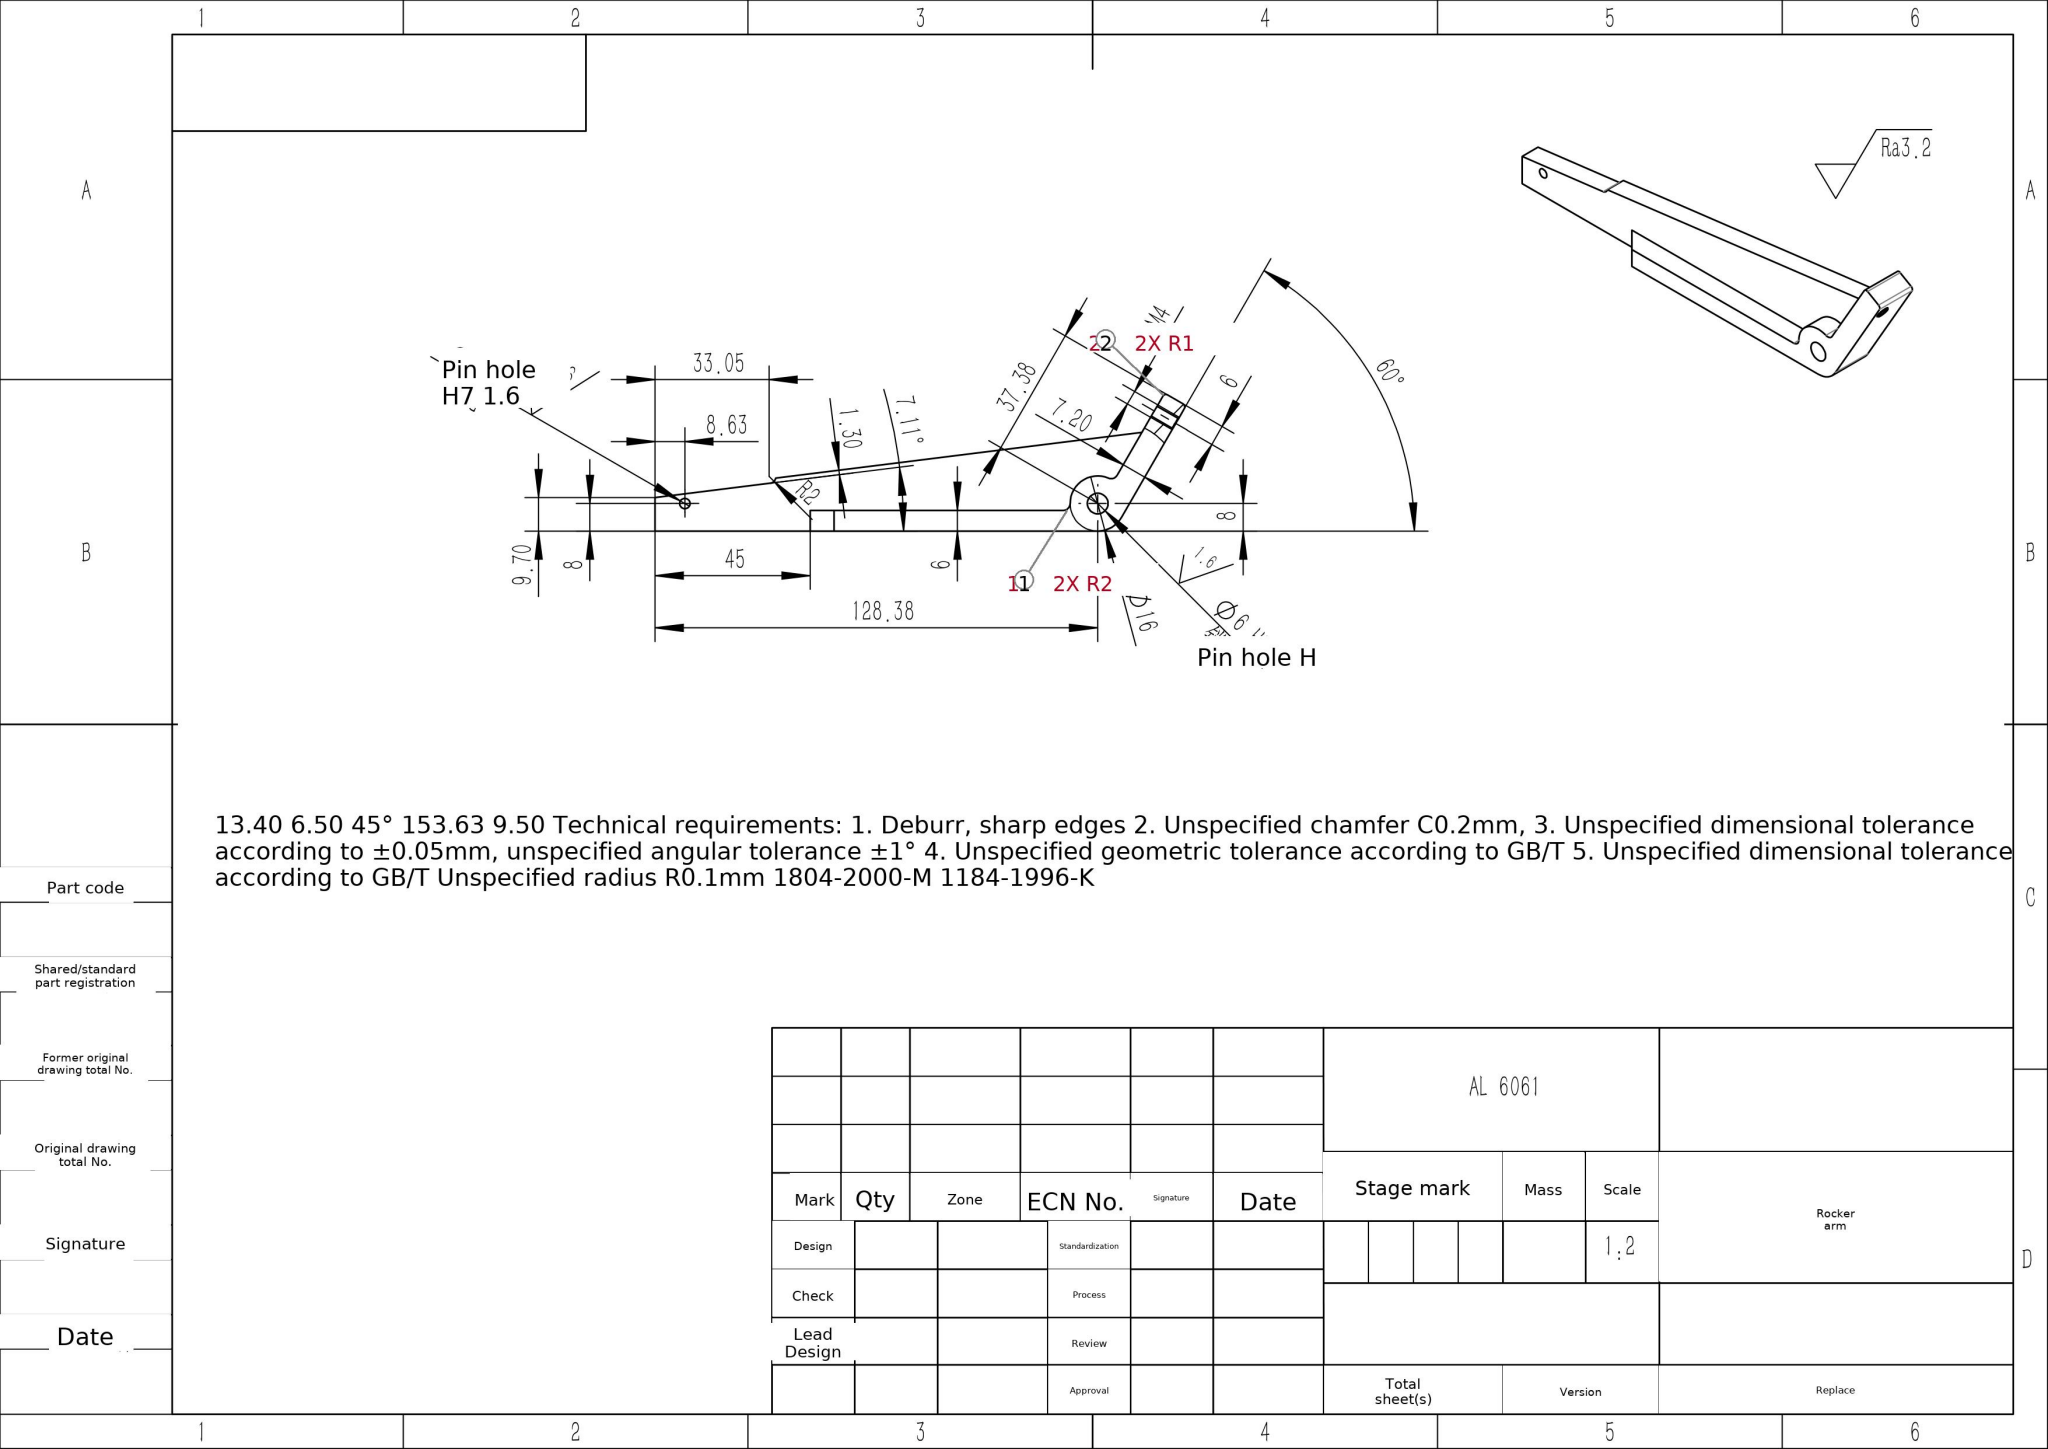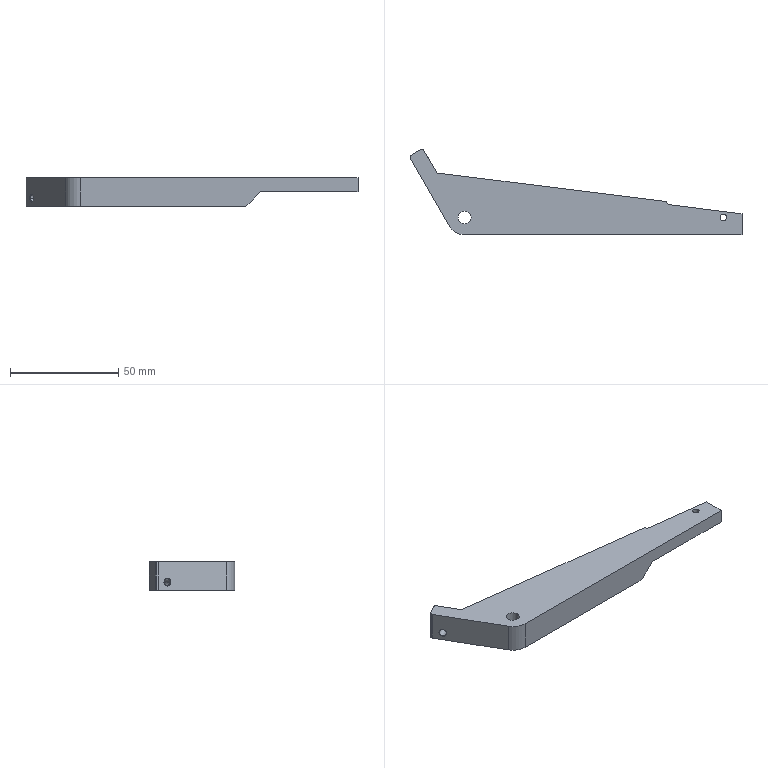Part | SolidWorks | mm | material AL 6061 | 1 solid | 28 faces | box 153.63 x 39.61 x 13.4 mm | volume 23931 mm3 | cylinder 14 | plane 12 | cone 2 | commonest cylinder face diameters 2 x3 4 x3 3.3 x2 6 x2 3 x2 16 x2
STEP:
#1=CARTESIAN_POINT('',(-89.039,32.706,-3.));
#2=VERTEX_POINT('',#1);
#3=CARTESIAN_POINT('',(-87.389,29.848,-3.));
#4=VERTEX_POINT('',#3);
#5=CARTESIAN_POINT('',(-88.214,31.277,-3.));
#6=DIRECTION('',(-0.866,-0.5,0.));
#7=DIRECTION('',(-0.5,0.866,0.));
#8=AXIS2_PLACEMENT_3D('',#5,#6,#7);
#9=CIRCLE('',#8,1.65);
#10=EDGE_CURVE('',#2,#4,#9,.T.);
#11=ORIENTED_EDGE('',*,*,#10,.F.);
#12=CARTESIAN_POINT('',(-89.312,32.779,-3.));
#13=VERTEX_POINT('',#12);
#14=CARTESIAN_POINT('',(-89.039,32.706,-3.));
#15=DIRECTION('',(-0.9659,0.2588,0.));
#16=VECTOR('',#15,1000.);
#17=LINE('',#14,#16);
#18=EDGE_CURVE('',#2,#13,#17,.T.);
#19=ORIENTED_EDGE('',*,*,#18,.T.);
#20=CARTESIAN_POINT('',(-87.462,29.575,-3.));
#21=VERTEX_POINT('',#20);
#22=CARTESIAN_POINT('',(-88.387,31.177,-3.));
#23=DIRECTION('',(0.866,0.5,0.));
#24=DIRECTION('',(-0.5,0.866,0.));
#25=AXIS2_PLACEMENT_3D('',#22,#23,#24);
#26=CIRCLE('',#25,1.85);
#27=EDGE_CURVE('',#21,#13,#26,.T.);
#28=ORIENTED_EDGE('',*,*,#27,.F.);
#29=CARTESIAN_POINT('',(-87.389,29.848,-3.));
#30=DIRECTION('',(-0.2588,-0.9659,0.));
#31=VECTOR('',#30,1000.);
#32=LINE('',#29,#31);
#33=EDGE_CURVE('',#4,#21,#32,.T.);
#34=ORIENTED_EDGE('',*,*,#33,.F.);
#35=EDGE_LOOP('',(#11,#19,#28,#34));
#36=FACE_OUTER_BOUND('',#35,.T.);
#37=CARTESIAN_POINT('',(-88.214,31.277,-3.));
#38=DIRECTION('',(-0.866,-0.5,0.));
#39=DIRECTION('',(0.5,-0.866,0.));
#40=AXIS2_PLACEMENT_3D('',#37,#38,#39);
#41=CONICAL_SURFACE('',#40,1.65,0.7854);
#42=ADVANCED_FACE('',(#36),#41,.F.);
#43=CARTESIAN_POINT('',(-82.976,36.206,-3.));
#44=VERTEX_POINT('',#43);
#45=CARTESIAN_POINT('',(-81.326,33.348,-3.));
#46=VERTEX_POINT('',#45);
#47=CARTESIAN_POINT('',(-82.151,34.777,-3.));
#48=DIRECTION('',(-0.866,-0.5,0.));
#49=DIRECTION('',(0.5,-0.866,0.));
#50=AXIS2_PLACEMENT_3D('',#47,#48,#49);
#51=CIRCLE('',#50,1.65);
#52=EDGE_CURVE('',#44,#46,#51,.T.);
#53=ORIENTED_EDGE('',*,*,#52,.F.);
#54=CARTESIAN_POINT('',(27.688,100.098,-3.));
#55=DIRECTION('',(-0.866,-0.5,0.));
#56=VECTOR('',#55,1000.);
#57=LINE('',#54,#56);
#58=EDGE_CURVE('',#44,#2,#57,.T.);
#59=ORIENTED_EDGE('',*,*,#58,.T.);
#60=ORIENTED_EDGE('',*,*,#10,.T.);
#61=CARTESIAN_POINT('',(29.338,97.24,-3.));
#62=DIRECTION('',(-0.866,-0.5,0.));
#63=VECTOR('',#62,1000.);
#64=LINE('',#61,#63);
#65=EDGE_CURVE('',#46,#4,#64,.T.);
#66=ORIENTED_EDGE('',*,*,#65,.F.);
#67=EDGE_LOOP('',(#53,#59,#60,#66));
#68=FACE_OUTER_BOUND('',#67,.T.);
#69=CARTESIAN_POINT('',(28.513,98.669,-3.));
#70=DIRECTION('',(-0.866,-0.5,0.));
#71=DIRECTION('',(0.5,-0.866,0.));
#72=AXIS2_PLACEMENT_3D('',#69,#70,#71);
#73=CYLINDRICAL_SURFACE('',#72,1.65);
#74=ADVANCED_FACE('',(#68),#73,.F.);
#75=CARTESIAN_POINT('',(-62.768,8.,-6.9));
#76=VERTEX_POINT('',#75);
#77=CARTESIAN_POINT('',(-68.768,8.,-6.9));
#78=VERTEX_POINT('',#77);
#79=CARTESIAN_POINT('',(-65.768,8.,-6.9));
#80=DIRECTION('',(0.,0.,-1.));
#81=DIRECTION('',(1.,0.,0.));
#82=AXIS2_PLACEMENT_3D('',#79,#80,#81);
#83=CIRCLE('',#82,3.);
#84=EDGE_CURVE('',#76,#78,#83,.T.);
#85=ORIENTED_EDGE('',*,*,#84,.T.);
#86=CARTESIAN_POINT('',(-68.768,8.,6.5));
#87=VERTEX_POINT('',#86);
#88=CARTESIAN_POINT('',(-68.768,8.,-15.485));
#89=DIRECTION('',(0.,0.,1.));
#90=VECTOR('',#89,1000.);
#91=LINE('',#88,#90);
#92=EDGE_CURVE('',#78,#87,#91,.T.);
#93=ORIENTED_EDGE('',*,*,#92,.T.);
#94=CARTESIAN_POINT('',(-62.768,8.,6.5));
#95=VERTEX_POINT('',#94);
#96=CARTESIAN_POINT('',(-65.768,8.,6.5));
#97=DIRECTION('',(0.,0.,1.));
#98=DIRECTION('',(1.,0.,0.));
#99=AXIS2_PLACEMENT_3D('',#96,#97,#98);
#100=CIRCLE('',#99,3.);
#101=EDGE_CURVE('',#87,#95,#100,.T.);
#102=ORIENTED_EDGE('',*,*,#101,.T.);
#103=CARTESIAN_POINT('',(-62.768,8.,-15.485));
#104=DIRECTION('',(0.,0.,1.));
#105=VECTOR('',#104,1000.);
#106=LINE('',#103,#105);
#107=EDGE_CURVE('',#76,#95,#106,.T.);
#108=ORIENTED_EDGE('',*,*,#107,.F.);
#109=EDGE_LOOP('',(#85,#93,#102,#108));
#110=FACE_OUTER_BOUND('',#109,.T.);
#111=CARTESIAN_POINT('',(-65.768,8.,-15.485));
#112=DIRECTION('',(0.,0.,1.));
#113=DIRECTION('',(1.,0.,0.));
#114=AXIS2_PLACEMENT_3D('',#111,#112,#113);
#115=CYLINDRICAL_SURFACE('',#114,3.);
#116=ADVANCED_FACE('',(#110),#115,.F.);
#117=CARTESIAN_POINT('',(-91.021,36.007,6.5));
#118=VERTEX_POINT('',#117);
#119=CARTESIAN_POINT('',(-90.887,35.507,6.5));
#120=VERTEX_POINT('',#119);
#121=CARTESIAN_POINT('',(-90.021,36.007,6.5));
#122=DIRECTION('',(0.,0.,1.));
#123=DIRECTION('',(1.,0.,0.));
#124=AXIS2_PLACEMENT_3D('',#121,#122,#123);
#125=CIRCLE('',#124,1.);
#126=EDGE_CURVE('',#118,#120,#125,.T.);
#127=ORIENTED_EDGE('',*,*,#126,.F.);
#128=CARTESIAN_POINT('',(-91.021,36.007,-6.9));
#129=VERTEX_POINT('',#128);
#130=CARTESIAN_POINT('',(-91.021,36.007,6.5));
#131=DIRECTION('',(0.,0.,-1.));
#132=VECTOR('',#131,1000.);
#133=LINE('',#130,#132);
#134=EDGE_CURVE('',#118,#129,#133,.T.);
#135=ORIENTED_EDGE('',*,*,#134,.T.);
#136=CARTESIAN_POINT('',(-90.887,35.507,-6.9));
#137=VERTEX_POINT('',#136);
#138=CARTESIAN_POINT('',(-90.021,36.007,-6.9));
#139=DIRECTION('',(0.,0.,1.));
#140=DIRECTION('',(1.,0.,0.));
#141=AXIS2_PLACEMENT_3D('',#138,#139,#140);
#142=CIRCLE('',#141,1.);
#143=EDGE_CURVE('',#129,#137,#142,.T.);
#144=ORIENTED_EDGE('',*,*,#143,.T.);
#145=CARTESIAN_POINT('',(-90.887,35.507,6.5));
#146=DIRECTION('',(0.,0.,-1.));
#147=VECTOR('',#146,1000.);
#148=LINE('',#145,#147);
#149=EDGE_CURVE('',#120,#137,#148,.T.);
#150=ORIENTED_EDGE('',*,*,#149,.F.);
#151=EDGE_LOOP('',(#127,#135,#144,#150));
#152=FACE_OUTER_BOUND('',#151,.T.);
#153=CARTESIAN_POINT('',(-90.021,36.007,6.5));
#154=DIRECTION('',(0.,0.,-1.));
#155=DIRECTION('',(-1.,0.,0.));
#156=AXIS2_PLACEMENT_3D('',#153,#154,#155);
#157=CYLINDRICAL_SURFACE('',#156,1.);
#158=ADVANCED_FACE('',(#152),#157,.T.);
#159=CARTESIAN_POINT('',(52.482,8.,0.));
#160=VERTEX_POINT('',#159);
#161=CARTESIAN_POINT('',(55.482,8.,0.));
#162=VERTEX_POINT('',#161);
#163=CARTESIAN_POINT('',(53.982,8.,0.));
#164=DIRECTION('',(0.,0.,1.));
#165=DIRECTION('',(1.,0.,0.));
#166=AXIS2_PLACEMENT_3D('',#163,#164,#165);
#167=CIRCLE('',#166,1.5);
#168=EDGE_CURVE('',#160,#162,#167,.T.);
#169=ORIENTED_EDGE('',*,*,#168,.F.);
#170=CARTESIAN_POINT('',(52.482,8.,6.5));
#171=VERTEX_POINT('',#170);
#172=CARTESIAN_POINT('',(52.482,8.,-0.5));
#173=DIRECTION('',(0.,0.,1.));
#174=VECTOR('',#173,1000.);
#175=LINE('',#172,#174);
#176=EDGE_CURVE('',#160,#171,#175,.T.);
#177=ORIENTED_EDGE('',*,*,#176,.T.);
#178=CARTESIAN_POINT('',(55.482,8.,6.5));
#179=VERTEX_POINT('',#178);
#180=CARTESIAN_POINT('',(53.982,8.,6.5));
#181=DIRECTION('',(0.,0.,1.));
#182=DIRECTION('',(1.,0.,0.));
#183=AXIS2_PLACEMENT_3D('',#180,#181,#182);
#184=CIRCLE('',#183,1.5);
#185=EDGE_CURVE('',#171,#179,#184,.T.);
#186=ORIENTED_EDGE('',*,*,#185,.T.);
#187=CARTESIAN_POINT('',(55.482,8.,-0.5));
#188=DIRECTION('',(0.,0.,1.));
#189=VECTOR('',#188,1000.);
#190=LINE('',#187,#189);
#191=EDGE_CURVE('',#162,#179,#190,.T.);
#192=ORIENTED_EDGE('',*,*,#191,.F.);
#193=EDGE_LOOP('',(#169,#177,#186,#192));
#194=FACE_OUTER_BOUND('',#193,.T.);
#195=CARTESIAN_POINT('',(53.982,8.,-0.5));
#196=DIRECTION('',(0.,0.,1.));
#197=DIRECTION('',(1.,0.,0.));
#198=AXIS2_PLACEMENT_3D('',#195,#196,#197);
#199=CYLINDRICAL_SURFACE('',#198,1.5);
#200=ADVANCED_FACE('',(#194),#199,.F.);
#201=CARTESIAN_POINT('',(-82.151,34.777,-3.));
#202=DIRECTION('',(-0.866,-0.5,0.));
#203=DIRECTION('',(0.5,-0.866,0.));
#204=AXIS2_PLACEMENT_3D('',#201,#202,#203);
#205=CIRCLE('',#204,1.65);
#206=EDGE_CURVE('',#46,#44,#205,.T.);
#207=ORIENTED_EDGE('',*,*,#206,.T.);
#208=ORIENTED_EDGE('',*,*,#52,.T.);
#209=EDGE_LOOP('',(#207,#208));
#210=FACE_BOUND('',#209,.T.);
#211=CARTESIAN_POINT('',(-71.425,16.198,0.));
#212=VERTEX_POINT('',#211);
#213=CARTESIAN_POINT('',(-71.425,16.198,-6.9));
#214=VERTEX_POINT('',#213);
#215=CARTESIAN_POINT('',(-71.425,16.198,-7.));
#216=DIRECTION('',(0.,0.,-1.));
#217=VECTOR('',#216,1000.);
#218=LINE('',#215,#217);
#219=EDGE_CURVE('',#212,#214,#218,.T.);
#220=ORIENTED_EDGE('',*,*,#219,.T.);
#221=CARTESIAN_POINT('',(-84.651,39.107,-6.9));
#222=VERTEX_POINT('',#221);
#223=CARTESIAN_POINT('',(-85.151,39.973,-6.9));
#224=DIRECTION('',(-0.5,0.866,0.));
#225=VECTOR('',#224,1000.);
#226=LINE('',#223,#225);
#227=EDGE_CURVE('',#214,#222,#226,.T.);
#228=ORIENTED_EDGE('',*,*,#227,.T.);
#229=CARTESIAN_POINT('',(-84.651,39.107,6.5));
#230=VERTEX_POINT('',#229);
#231=CARTESIAN_POINT('',(-84.651,39.107,6.5));
#232=DIRECTION('',(0.,0.,1.));
#233=VECTOR('',#232,1000.);
#234=LINE('',#231,#233);
#235=EDGE_CURVE('',#222,#230,#234,.T.);
#236=ORIENTED_EDGE('',*,*,#235,.T.);
#237=CARTESIAN_POINT('',(-78.598,28.621,6.5));
#238=VERTEX_POINT('',#237);
#239=CARTESIAN_POINT('',(-85.151,39.973,6.5));
#240=DIRECTION('',(-0.5,0.866,0.));
#241=VECTOR('',#240,1000.);
#242=LINE('',#239,#241);
#243=EDGE_CURVE('',#238,#230,#242,.T.);
#244=ORIENTED_EDGE('',*,*,#243,.F.);
#245=CARTESIAN_POINT('',(-78.598,28.621,0.));
#246=VERTEX_POINT('',#245);
#247=CARTESIAN_POINT('',(-78.598,28.621,6.5));
#248=DIRECTION('',(-0.,-0.,-1.));
#249=VECTOR('',#248,1000.);
#250=LINE('',#247,#249);
#251=EDGE_CURVE('',#238,#246,#250,.T.);
#252=ORIENTED_EDGE('',*,*,#251,.T.);
#253=CARTESIAN_POINT('',(-46.555,-26.878,0.));
#254=DIRECTION('',(0.5,-0.866,0.));
#255=VECTOR('',#254,1000.);
#256=LINE('',#253,#255);
#257=EDGE_CURVE('',#246,#212,#256,.T.);
#258=ORIENTED_EDGE('',*,*,#257,.T.);
#259=EDGE_LOOP('',(#220,#228,#236,#244,#252,#258));
#260=FACE_OUTER_BOUND('',#259,.T.);
#261=CARTESIAN_POINT('',(-85.151,39.973,6.5));
#262=DIRECTION('',(-0.866,-0.5,0.));
#263=DIRECTION('',(0.5,-0.866,0.));
#264=AXIS2_PLACEMENT_3D('',#261,#262,#263);
#265=PLANE('',#264);
#266=ADVANCED_FACE('',(#210,#260),#265,.F.);
#267=CARTESIAN_POINT('',(-55.768,6.,-6.9));
#268=VERTEX_POINT('',#267);
#269=CARTESIAN_POINT('',(-55.768,6.,0.));
#270=VERTEX_POINT('',#269);
#271=CARTESIAN_POINT('',(-55.768,6.,0.));
#272=DIRECTION('',(0.,0.,1.));
#273=VECTOR('',#272,1000.);
#274=LINE('',#271,#273);
#275=EDGE_CURVE('',#268,#270,#274,.T.);
#276=ORIENTED_EDGE('',*,*,#275,.T.);
#277=CARTESIAN_POINT('',(17.613,6.,0.));
#278=VERTEX_POINT('',#277);
#279=CARTESIAN_POINT('',(-0.,6.,0.));
#280=DIRECTION('',(1.,0.,0.));
#281=VECTOR('',#280,1000.);
#282=LINE('',#279,#281);
#283=EDGE_CURVE('',#270,#278,#282,.T.);
#284=ORIENTED_EDGE('',*,*,#283,.T.);
#285=CARTESIAN_POINT('',(10.713,6.,-6.9));
#286=VERTEX_POINT('',#285);
#287=CARTESIAN_POINT('',(10.613,6.,-7.));
#288=DIRECTION('',(-0.7071,-0.,-0.7071));
#289=VECTOR('',#288,1000.);
#290=LINE('',#287,#289);
#291=EDGE_CURVE('',#278,#286,#290,.T.);
#292=ORIENTED_EDGE('',*,*,#291,.T.);
#293=CARTESIAN_POINT('',(-0.,6.,-6.9));
#294=DIRECTION('',(1.,0.,0.));
#295=VECTOR('',#294,1000.);
#296=LINE('',#293,#295);
#297=EDGE_CURVE('',#268,#286,#296,.T.);
#298=ORIENTED_EDGE('',*,*,#297,.F.);
#299=EDGE_LOOP('',(#276,#284,#292,#298));
#300=FACE_OUTER_BOUND('',#299,.T.);
#301=CARTESIAN_POINT('',(17.613,6.,-7.));
#302=DIRECTION('',(0.,-1.,0.));
#303=DIRECTION('',(1.,0.,0.));
#304=AXIS2_PLACEMENT_3D('',#301,#302,#303);
#305=PLANE('',#304);
#306=ADVANCED_FACE('',(#300),#305,.F.);
#307=CARTESIAN_POINT('',(53.982,8.,0.));
#308=DIRECTION('',(0.,0.,1.));
#309=DIRECTION('',(1.,0.,0.));
#310=AXIS2_PLACEMENT_3D('',#307,#308,#309);
#311=CIRCLE('',#310,1.5);
#312=EDGE_CURVE('',#162,#160,#311,.T.);
#313=ORIENTED_EDGE('',*,*,#312,.T.);
#314=ORIENTED_EDGE('',*,*,#168,.T.);
#315=EDGE_LOOP('',(#313,#314));
#316=FACE_BOUND('',#315,.T.);
#317=CARTESIAN_POINT('',(17.613,0.,0.));
#318=VERTEX_POINT('',#317);
#319=CARTESIAN_POINT('',(17.613,-0.,0.));
#320=DIRECTION('',(0.,-1.,0.));
#321=VECTOR('',#320,1000.);
#322=LINE('',#319,#321);
#323=EDGE_CURVE('',#278,#318,#322,.T.);
#324=ORIENTED_EDGE('',*,*,#323,.F.);
#325=ORIENTED_EDGE('',*,*,#283,.F.);
#326=CARTESIAN_POINT('',(-57.768,8.,0.));
#327=VERTEX_POINT('',#326);
#328=CARTESIAN_POINT('',(-55.768,8.,0.));
#329=DIRECTION('',(0.,0.,1.));
#330=DIRECTION('',(1.,0.,0.));
#331=AXIS2_PLACEMENT_3D('',#328,#329,#330);
#332=CIRCLE('',#331,2.);
#333=EDGE_CURVE('',#327,#270,#332,.T.);
#334=ORIENTED_EDGE('',*,*,#333,.F.);
#335=CARTESIAN_POINT('',(-68.908,15.358,0.));
#336=VERTEX_POINT('',#335);
#337=CARTESIAN_POINT('',(-65.768,8.,0.));
#338=DIRECTION('',(0.,0.,-1.));
#339=DIRECTION('',(1.,0.,0.));
#340=AXIS2_PLACEMENT_3D('',#337,#338,#339);
#341=CIRCLE('',#340,8.);
#342=EDGE_CURVE('',#336,#327,#341,.T.);
#343=ORIENTED_EDGE('',*,*,#342,.F.);
#344=CARTESIAN_POINT('',(-69.693,17.198,0.));
#345=DIRECTION('',(0.,0.,1.));
#346=DIRECTION('',(1.,0.,0.));
#347=AXIS2_PLACEMENT_3D('',#344,#345,#346);
#348=CIRCLE('',#347,2.);
#349=EDGE_CURVE('',#212,#336,#348,.T.);
#350=ORIENTED_EDGE('',*,*,#349,.F.);
#351=ORIENTED_EDGE('',*,*,#257,.F.);
#352=CARTESIAN_POINT('',(27.613,15.376,0.));
#353=VERTEX_POINT('',#352);
#354=CARTESIAN_POINT('',(27.904,15.339,-0.));
#355=DIRECTION('',(-0.9923,0.1238,0.));
#356=VECTOR('',#355,1000.);
#357=LINE('',#354,#356);
#358=EDGE_CURVE('',#353,#246,#357,.T.);
#359=ORIENTED_EDGE('',*,*,#358,.F.);
#360=CARTESIAN_POINT('',(29.311,13.854,-0.));
#361=VERTEX_POINT('',#360);
#362=CARTESIAN_POINT('',(29.559,15.838,0.));
#363=DIRECTION('',(0.,0.,1.));
#364=DIRECTION('',(1.,0.,0.));
#365=AXIS2_PLACEMENT_3D('',#362,#363,#364);
#366=CIRCLE('',#365,2.);
#367=EDGE_CURVE('',#353,#361,#366,.T.);
#368=ORIENTED_EDGE('',*,*,#367,.T.);
#369=CARTESIAN_POINT('',(62.613,9.701,0.));
#370=VERTEX_POINT('',#369);
#371=CARTESIAN_POINT('',(28.189,13.994,-0.));
#372=DIRECTION('',(-0.9923,0.1238,0.));
#373=VECTOR('',#372,1000.);
#374=LINE('',#371,#373);
#375=EDGE_CURVE('',#370,#361,#374,.T.);
#376=ORIENTED_EDGE('',*,*,#375,.F.);
#377=CARTESIAN_POINT('',(62.613,0.,0.));
#378=VERTEX_POINT('',#377);
#379=CARTESIAN_POINT('',(62.613,0.,0.));
#380=DIRECTION('',(0.,1.,0.));
#381=VECTOR('',#380,1000.);
#382=LINE('',#379,#381);
#383=EDGE_CURVE('',#378,#370,#382,.T.);
#384=ORIENTED_EDGE('',*,*,#383,.F.);
#385=CARTESIAN_POINT('',(62.613,0.,0.));
#386=DIRECTION('',(1.,0.,0.));
#387=VECTOR('',#386,1000.);
#388=LINE('',#385,#387);
#389=EDGE_CURVE('',#318,#378,#388,.T.);
#390=ORIENTED_EDGE('',*,*,#389,.F.);
#391=EDGE_LOOP('',(#324,#325,#334,#343,#350,#351,#359,#368,#376,#384,#390));
#392=FACE_OUTER_BOUND('',#391,.T.);
#393=CARTESIAN_POINT('',(0.,0.,0.));
#394=DIRECTION('',(0.,0.,1.));
#395=DIRECTION('',(1.,0.,0.));
#396=AXIS2_PLACEMENT_3D('',#393,#394,#395);
#397=PLANE('',#396);
#398=ADVANCED_FACE('',(#316,#392),#397,.F.);
#399=ORIENTED_EDGE('',*,*,#383,.T.);
#400=CARTESIAN_POINT('',(62.613,9.701,6.5));
#401=VERTEX_POINT('',#400);
#402=CARTESIAN_POINT('',(62.613,9.701,6.5));
#403=DIRECTION('',(0.,-0.,-1.));
#404=VECTOR('',#403,1000.);
#405=LINE('',#402,#404);
#406=EDGE_CURVE('',#401,#370,#405,.T.);
#407=ORIENTED_EDGE('',*,*,#406,.F.);
#408=CARTESIAN_POINT('',(62.613,0.,6.5));
#409=VERTEX_POINT('',#408);
#410=CARTESIAN_POINT('',(62.613,0.,6.5));
#411=DIRECTION('',(0.,1.,0.));
#412=VECTOR('',#411,1000.);
#413=LINE('',#410,#412);
#414=EDGE_CURVE('',#409,#401,#413,.T.);
#415=ORIENTED_EDGE('',*,*,#414,.F.);
#416=CARTESIAN_POINT('',(62.613,0.,6.5));
#417=DIRECTION('',(0.,0.,-1.));
#418=VECTOR('',#417,1000.);
#419=LINE('',#416,#418);
#420=EDGE_CURVE('',#409,#378,#419,.T.);
#421=ORIENTED_EDGE('',*,*,#420,.T.);
#422=EDGE_LOOP('',(#399,#407,#415,#421));
#423=FACE_OUTER_BOUND('',#422,.T.);
#424=CARTESIAN_POINT('',(62.613,0.,6.5));
#425=DIRECTION('',(-1.,0.,0.));
#426=DIRECTION('',(0.,0.,1.));
#427=AXIS2_PLACEMENT_3D('',#424,#425,#426);
#428=PLANE('',#427);
#429=ADVANCED_FACE('',(#423),#428,.F.);
#430=ORIENTED_EDGE('',*,*,#375,.T.);
#431=CARTESIAN_POINT('',(29.311,13.854,6.5));
#432=VERTEX_POINT('',#431);
#433=CARTESIAN_POINT('',(29.311,13.854,6.5));
#434=DIRECTION('',(0.,0.,1.));
#435=VECTOR('',#434,1000.);
#436=LINE('',#433,#435);
#437=EDGE_CURVE('',#361,#432,#436,.T.);
#438=ORIENTED_EDGE('',*,*,#437,.T.);
#439=CARTESIAN_POINT('',(28.189,13.994,6.5));
#440=DIRECTION('',(-0.9923,0.1238,0.));
#441=VECTOR('',#440,1000.);
#442=LINE('',#439,#441);
#443=EDGE_CURVE('',#401,#432,#442,.T.);
#444=ORIENTED_EDGE('',*,*,#443,.F.);
#445=ORIENTED_EDGE('',*,*,#406,.T.);
#446=EDGE_LOOP('',(#430,#438,#444,#445));
#447=FACE_OUTER_BOUND('',#446,.T.);
#448=CARTESIAN_POINT('',(28.189,13.994,6.5));
#449=DIRECTION('',(-0.1238,-0.9923,0.));
#450=DIRECTION('',(0.9923,-0.1238,-0.));
#451=AXIS2_PLACEMENT_3D('',#448,#449,#450);
#452=PLANE('',#451);
#453=ADVANCED_FACE('',(#447),#452,.F.);
#454=ORIENTED_EDGE('',*,*,#358,.T.);
#455=ORIENTED_EDGE('',*,*,#251,.F.);
#456=CARTESIAN_POINT('',(27.613,15.376,6.5));
#457=VERTEX_POINT('',#456);
#458=CARTESIAN_POINT('',(27.904,15.339,6.5));
#459=DIRECTION('',(-0.9923,0.1238,0.));
#460=VECTOR('',#459,1000.);
#461=LINE('',#458,#460);
#462=EDGE_CURVE('',#457,#238,#461,.T.);
#463=ORIENTED_EDGE('',*,*,#462,.F.);
#464=CARTESIAN_POINT('',(27.613,15.376,6.5));
#465=DIRECTION('',(0.,-0.,-1.));
#466=VECTOR('',#465,1000.);
#467=LINE('',#464,#466);
#468=EDGE_CURVE('',#457,#353,#467,.T.);
#469=ORIENTED_EDGE('',*,*,#468,.T.);
#470=EDGE_LOOP('',(#454,#455,#463,#469));
#471=FACE_OUTER_BOUND('',#470,.T.);
#472=CARTESIAN_POINT('',(27.904,15.339,6.5));
#473=DIRECTION('',(-0.1238,-0.9923,0.));
#474=DIRECTION('',(0.9923,-0.1238,-0.));
#475=AXIS2_PLACEMENT_3D('',#472,#473,#474);
#476=PLANE('',#475);
#477=ADVANCED_FACE('',(#471),#476,.F.);
#478=CARTESIAN_POINT('',(-86.018,39.473,6.5));
#479=VERTEX_POINT('',#478);
#480=CARTESIAN_POINT('',(-86.018,39.473,-6.9));
#481=VERTEX_POINT('',#480);
#482=CARTESIAN_POINT('',(-86.018,39.473,6.5));
#483=DIRECTION('',(0.,0.,-1.));
#484=VECTOR('',#483,1000.);
#485=LINE('',#482,#484);
#486=EDGE_CURVE('',#479,#481,#485,.T.);
#487=ORIENTED_EDGE('',*,*,#486,.T.);
#488=CARTESIAN_POINT('',(-90.521,36.873,-6.9));
#489=VERTEX_POINT('',#488);
#490=CARTESIAN_POINT('',(-91.387,36.373,-6.9));
#491=DIRECTION('',(-0.866,-0.5,0.));
#492=VECTOR('',#491,1000.);
#493=LINE('',#490,#492);
#494=EDGE_CURVE('',#481,#489,#493,.T.);
#495=ORIENTED_EDGE('',*,*,#494,.T.);
#496=CARTESIAN_POINT('',(-90.521,36.873,6.5));
#497=VERTEX_POINT('',#496);
#498=CARTESIAN_POINT('',(-90.521,36.873,6.5));
#499=DIRECTION('',(0.,0.,1.));
#500=VECTOR('',#499,1000.);
#501=LINE('',#498,#500);
#502=EDGE_CURVE('',#489,#497,#501,.T.);
#503=ORIENTED_EDGE('',*,*,#502,.T.);
#504=CARTESIAN_POINT('',(-91.387,36.373,6.5));
#505=DIRECTION('',(-0.866,-0.5,0.));
#506=VECTOR('',#505,1000.);
#507=LINE('',#504,#506);
#508=EDGE_CURVE('',#479,#497,#507,.T.);
#509=ORIENTED_EDGE('',*,*,#508,.F.);
#510=EDGE_LOOP('',(#487,#495,#503,#509));
#511=FACE_OUTER_BOUND('',#510,.T.);
#512=CARTESIAN_POINT('',(-91.387,36.373,6.5));
#513=DIRECTION('',(0.5,-0.866,0.));
#514=DIRECTION('',(0.866,0.5,0.));
#515=AXIS2_PLACEMENT_3D('',#512,#513,#514);
#516=PLANE('',#515);
#517=ADVANCED_FACE('',(#511),#516,.F.);
#518=ORIENTED_EDGE('',*,*,#27,.T.);
#519=CARTESIAN_POINT('',(-88.387,31.177,-3.));
#520=DIRECTION('',(0.866,0.5,0.));
#521=DIRECTION('',(-0.5,0.866,0.));
#522=AXIS2_PLACEMENT_3D('',#519,#520,#521);
#523=CIRCLE('',#522,1.85);
#524=EDGE_CURVE('',#13,#21,#523,.T.);
#525=ORIENTED_EDGE('',*,*,#524,.T.);
#526=EDGE_LOOP('',(#518,#525));
#527=FACE_BOUND('',#526,.T.);
#528=ORIENTED_EDGE('',*,*,#149,.T.);
#529=CARTESIAN_POINT('',(-72.696,4.,-6.9));
#530=VERTEX_POINT('',#529);
#531=CARTESIAN_POINT('',(-70.387,0.,-6.9));
#532=DIRECTION('',(0.5,-0.866,0.));
#533=VECTOR('',#532,1000.);
#534=LINE('',#531,#533);
#535=EDGE_CURVE('',#137,#530,#534,.T.);
#536=ORIENTED_EDGE('',*,*,#535,.T.);
#537=CARTESIAN_POINT('',(-72.696,4.,6.5));
#538=VERTEX_POINT('',#537);
#539=CARTESIAN_POINT('',(-72.696,4.,6.5));
#540=DIRECTION('',(0.,0.,1.));
#541=VECTOR('',#540,1000.);
#542=LINE('',#539,#541);
#543=EDGE_CURVE('',#530,#538,#542,.T.);
#544=ORIENTED_EDGE('',*,*,#543,.T.);
#545=CARTESIAN_POINT('',(-70.387,0.,6.5));
#546=DIRECTION('',(0.5,-0.866,0.));
#547=VECTOR('',#546,1000.);
#548=LINE('',#545,#547);
#549=EDGE_CURVE('',#120,#538,#548,.T.);
#550=ORIENTED_EDGE('',*,*,#549,.F.);
#551=EDGE_LOOP('',(#528,#536,#544,#550));
#552=FACE_OUTER_BOUND('',#551,.T.);
#553=CARTESIAN_POINT('',(-70.387,0.,6.5));
#554=DIRECTION('',(0.866,0.5,0.));
#555=DIRECTION('',(-0.5,0.866,0.));
#556=AXIS2_PLACEMENT_3D('',#553,#554,#555);
#557=PLANE('',#556);
#558=ADVANCED_FACE('',(#527,#552),#557,.F.);
#559=CARTESIAN_POINT('',(-65.768,0.,6.5));
#560=VERTEX_POINT('',#559);
#561=CARTESIAN_POINT('',(-65.768,0.,-6.9));
#562=VERTEX_POINT('',#561);
#563=CARTESIAN_POINT('',(-65.768,0.,6.5));
#564=DIRECTION('',(0.,0.,-1.));
#565=VECTOR('',#564,1000.);
#566=LINE('',#563,#565);
#567=EDGE_CURVE('',#560,#562,#566,.T.);
#568=ORIENTED_EDGE('',*,*,#567,.T.);
#569=CARTESIAN_POINT('',(10.713,0.,-6.9));
#570=VERTEX_POINT('',#569);
#571=CARTESIAN_POINT('',(0.,0.,-6.9));
#572=DIRECTION('',(-1.,0.,0.));
#573=VECTOR('',#572,1000.);
#574=LINE('',#571,#573);
#575=EDGE_CURVE('',#570,#562,#574,.T.);
#576=ORIENTED_EDGE('',*,*,#575,.F.);
#577=CARTESIAN_POINT('',(10.613,0.,-7.));
#578=DIRECTION('',(0.7071,0.,0.7071));
#579=VECTOR('',#578,1000.);
#580=LINE('',#577,#579);
#581=EDGE_CURVE('',#570,#318,#580,.T.);
#582=ORIENTED_EDGE('',*,*,#581,.T.);
#583=ORIENTED_EDGE('',*,*,#389,.T.);
#584=ORIENTED_EDGE('',*,*,#420,.F.);
#585=CARTESIAN_POINT('',(62.613,0.,6.5));
#586=DIRECTION('',(1.,0.,0.));
#587=VECTOR('',#586,1000.);
#588=LINE('',#585,#587);
#589=EDGE_CURVE('',#560,#409,#588,.T.);
#590=ORIENTED_EDGE('',*,*,#589,.F.);
#591=EDGE_LOOP('',(#568,#576,#582,#583,#584,#590));
#592=FACE_OUTER_BOUND('',#591,.T.);
#593=CARTESIAN_POINT('',(62.613,0.,6.5));
#594=DIRECTION('',(0.,1.,0.));
#595=DIRECTION('',(0.,0.,1.));
#596=AXIS2_PLACEMENT_3D('',#593,#594,#595);
#597=PLANE('',#596);
#598=ADVANCED_FACE('',(#592),#597,.F.);
#599=CARTESIAN_POINT('',(-65.768,8.,6.5));
#600=DIRECTION('',(0.,0.,1.));
#601=DIRECTION('',(1.,0.,0.));
#602=AXIS2_PLACEMENT_3D('',#599,#600,#601);
#603=CIRCLE('',#602,3.);
#604=EDGE_CURVE('',#95,#87,#603,.T.);
#605=ORIENTED_EDGE('',*,*,#604,.F.);
#606=ORIENTED_EDGE('',*,*,#101,.F.);
#607=EDGE_LOOP('',(#605,#606));
#608=FACE_BOUND('',#607,.T.);
#609=CARTESIAN_POINT('',(53.982,8.,6.5));
#610=DIRECTION('',(0.,0.,1.));
#611=DIRECTION('',(1.,0.,0.));
#612=AXIS2_PLACEMENT_3D('',#609,#610,#611);
#613=CIRCLE('',#612,1.5);
#614=EDGE_CURVE('',#179,#171,#613,.T.);
#615=ORIENTED_EDGE('',*,*,#614,.F.);
#616=ORIENTED_EDGE('',*,*,#185,.F.);
#617=EDGE_LOOP('',(#615,#616));
#618=FACE_BOUND('',#617,.T.);
#619=ORIENTED_EDGE('',*,*,#508,.T.);
#620=CARTESIAN_POINT('',(-90.021,36.007,6.5));
#621=DIRECTION('',(0.,0.,1.));
#622=DIRECTION('',(1.,0.,0.));
#623=AXIS2_PLACEMENT_3D('',#620,#621,#622);
#624=CIRCLE('',#623,1.);
#625=EDGE_CURVE('',#497,#118,#624,.T.);
#626=ORIENTED_EDGE('',*,*,#625,.T.);
#627=ORIENTED_EDGE('',*,*,#126,.T.);
#628=ORIENTED_EDGE('',*,*,#549,.T.);
#629=CARTESIAN_POINT('',(-65.768,8.,6.5));
#630=DIRECTION('',(0.,0.,1.));
#631=DIRECTION('',(1.,0.,0.));
#632=AXIS2_PLACEMENT_3D('',#629,#630,#631);
#633=CIRCLE('',#632,8.);
#634=EDGE_CURVE('',#538,#560,#633,.T.);
#635=ORIENTED_EDGE('',*,*,#634,.T.);
#636=ORIENTED_EDGE('',*,*,#589,.T.);
#637=ORIENTED_EDGE('',*,*,#414,.T.);
#638=ORIENTED_EDGE('',*,*,#443,.T.);
#639=CARTESIAN_POINT('',(29.559,15.838,6.5));
#640=DIRECTION('',(0.,0.,-1.));
#641=DIRECTION('',(1.,0.,0.));
#642=AXIS2_PLACEMENT_3D('',#639,#640,#641);
#643=CIRCLE('',#642,2.);
#644=EDGE_CURVE('',#432,#457,#643,.T.);
#645=ORIENTED_EDGE('',*,*,#644,.T.);
#646=ORIENTED_EDGE('',*,*,#462,.T.);
#647=ORIENTED_EDGE('',*,*,#243,.T.);
#648=CARTESIAN_POINT('',(-85.518,38.607,6.5));
#649=DIRECTION('',(0.,0.,1.));
#650=DIRECTION('',(1.,0.,0.));
#651=AXIS2_PLACEMENT_3D('',#648,#649,#650);
#652=CIRCLE('',#651,1.);
#653=EDGE_CURVE('',#230,#479,#652,.T.);
#654=ORIENTED_EDGE('',*,*,#653,.T.);
#655=EDGE_LOOP('',(#619,#626,#627,#628,#635,#636,#637,#638,#645,#646,#647,#654));
#656=FACE_OUTER_BOUND('',#655,.T.);
#657=CARTESIAN_POINT('',(0.,0.,6.5));
#658=DIRECTION('',(0.,0.,1.));
#659=DIRECTION('',(1.,0.,0.));
#660=AXIS2_PLACEMENT_3D('',#657,#658,#659);
#661=PLANE('',#660);
#662=ADVANCED_FACE('',(#608,#618,#656),#661,.T.);
#663=ORIENTED_EDGE('',*,*,#84,.F.);
#664=CARTESIAN_POINT('',(-65.768,8.,-6.9));
#665=DIRECTION('',(0.,0.,-1.));
#666=DIRECTION('',(1.,0.,0.));
#667=AXIS2_PLACEMENT_3D('',#664,#665,#666);
#668=CIRCLE('',#667,3.);
#669=EDGE_CURVE('',#78,#76,#668,.T.);
#670=ORIENTED_EDGE('',*,*,#669,.F.);
#671=EDGE_LOOP('',(#663,#670));
#672=FACE_BOUND('',#671,.T.);
#673=ORIENTED_EDGE('',*,*,#575,.T.);
#674=CARTESIAN_POINT('',(-65.768,8.,-6.9));
#675=DIRECTION('',(0.,0.,-1.));
#676=DIRECTION('',(1.,0.,0.));
#677=AXIS2_PLACEMENT_3D('',#674,#675,#676);
#678=CIRCLE('',#677,8.);
#679=EDGE_CURVE('',#562,#530,#678,.T.);
#680=ORIENTED_EDGE('',*,*,#679,.T.);
#681=ORIENTED_EDGE('',*,*,#535,.F.);
#682=ORIENTED_EDGE('',*,*,#143,.F.);
#683=CARTESIAN_POINT('',(-90.021,36.007,-6.9));
#684=DIRECTION('',(0.,0.,1.));
#685=DIRECTION('',(1.,0.,0.));
#686=AXIS2_PLACEMENT_3D('',#683,#684,#685);
#687=CIRCLE('',#686,1.);
#688=EDGE_CURVE('',#489,#129,#687,.T.);
#689=ORIENTED_EDGE('',*,*,#688,.F.);
#690=ORIENTED_EDGE('',*,*,#494,.F.);
#691=CARTESIAN_POINT('',(-85.518,38.607,-6.9));
#692=DIRECTION('',(0.,0.,1.));
#693=DIRECTION('',(1.,0.,0.));
#694=AXIS2_PLACEMENT_3D('',#691,#692,#693);
#695=CIRCLE('',#694,1.);
#696=EDGE_CURVE('',#222,#481,#695,.T.);
#697=ORIENTED_EDGE('',*,*,#696,.F.);
#698=ORIENTED_EDGE('',*,*,#227,.F.);
#699=CARTESIAN_POINT('',(-68.908,15.358,-6.9));
#700=VERTEX_POINT('',#699);
#701=CARTESIAN_POINT('',(-69.693,17.198,-6.9));
#702=DIRECTION('',(0.,0.,1.));
#703=DIRECTION('',(1.,0.,0.));
#704=AXIS2_PLACEMENT_3D('',#701,#702,#703);
#705=CIRCLE('',#704,2.);
#706=EDGE_CURVE('',#214,#700,#705,.T.);
#707=ORIENTED_EDGE('',*,*,#706,.T.);
#708=CARTESIAN_POINT('',(-57.768,8.,-6.9));
#709=VERTEX_POINT('',#708);
#710=CARTESIAN_POINT('',(-65.768,8.,-6.9));
#711=DIRECTION('',(0.,0.,-1.));
#712=DIRECTION('',(1.,0.,0.));
#713=AXIS2_PLACEMENT_3D('',#710,#711,#712);
#714=CIRCLE('',#713,8.);
#715=EDGE_CURVE('',#700,#709,#714,.T.);
#716=ORIENTED_EDGE('',*,*,#715,.T.);
#717=CARTESIAN_POINT('',(-55.768,8.,-6.9));
#718=DIRECTION('',(0.,0.,1.));
#719=DIRECTION('',(1.,0.,0.));
#720=AXIS2_PLACEMENT_3D('',#717,#718,#719);
#721=CIRCLE('',#720,2.);
#722=EDGE_CURVE('',#709,#268,#721,.T.);
#723=ORIENTED_EDGE('',*,*,#722,.T.);
#724=ORIENTED_EDGE('',*,*,#297,.T.);
#725=CARTESIAN_POINT('',(10.713,0.,-6.9));
#726=DIRECTION('',(0.,-1.,0.));
#727=VECTOR('',#726,1000.);
#728=LINE('',#725,#727);
#729=EDGE_CURVE('',#286,#570,#728,.T.);
#730=ORIENTED_EDGE('',*,*,#729,.T.);
#731=EDGE_LOOP('',(#673,#680,#681,#682,#689,#690,#697,#698,#707,#716,#723,#724,#730));
#732=FACE_OUTER_BOUND('',#731,.T.);
#733=CARTESIAN_POINT('',(0.,0.,-6.9));
#734=DIRECTION('',(0.,0.,1.));
#735=DIRECTION('',(1.,0.,0.));
#736=AXIS2_PLACEMENT_3D('',#733,#734,#735);
#737=PLANE('',#736);
#738=ADVANCED_FACE('',(#672,#732),#737,.F.);
#739=CARTESIAN_POINT('',(-68.908,15.358,-29.627));
#740=DIRECTION('',(0.,0.,1.));
#741=VECTOR('',#740,1000.);
#742=LINE('',#739,#741);
#743=EDGE_CURVE('',#700,#336,#742,.T.);
#744=ORIENTED_EDGE('',*,*,#743,.T.);
#745=ORIENTED_EDGE('',*,*,#342,.T.);
#746=CARTESIAN_POINT('',(-57.768,8.,-29.627));
#747=DIRECTION('',(0.,0.,-1.));
#748=VECTOR('',#747,1000.);
#749=LINE('',#746,#748);
#750=EDGE_CURVE('',#327,#709,#749,.T.);
#751=ORIENTED_EDGE('',*,*,#750,.T.);
#752=ORIENTED_EDGE('',*,*,#715,.F.);
#753=EDGE_LOOP('',(#744,#745,#751,#752));
#754=FACE_OUTER_BOUND('',#753,.T.);
#755=CARTESIAN_POINT('',(-65.768,8.,-29.627));
#756=DIRECTION('',(0.,0.,1.));
#757=DIRECTION('',(1.,0.,0.));
#758=AXIS2_PLACEMENT_3D('',#755,#756,#757);
#759=CYLINDRICAL_SURFACE('',#758,8.);
#760=ADVANCED_FACE('',(#754),#759,.T.);
#761=ORIENTED_EDGE('',*,*,#543,.F.);
#762=ORIENTED_EDGE('',*,*,#679,.F.);
#763=ORIENTED_EDGE('',*,*,#567,.F.);
#764=ORIENTED_EDGE('',*,*,#634,.F.);
#765=EDGE_LOOP('',(#761,#762,#763,#764));
#766=FACE_OUTER_BOUND('',#765,.T.);
#767=CARTESIAN_POINT('',(-65.768,8.,6.5));
#768=DIRECTION('',(0.,0.,-1.));
#769=DIRECTION('',(-1.,0.,0.));
#770=AXIS2_PLACEMENT_3D('',#767,#768,#769);
#771=CYLINDRICAL_SURFACE('',#770,8.);
#772=ADVANCED_FACE('',(#766),#771,.T.);
#773=ORIENTED_EDGE('',*,*,#750,.F.);
#774=ORIENTED_EDGE('',*,*,#333,.T.);
#775=ORIENTED_EDGE('',*,*,#275,.F.);
#776=ORIENTED_EDGE('',*,*,#722,.F.);
#777=EDGE_LOOP('',(#773,#774,#775,#776));
#778=FACE_OUTER_BOUND('',#777,.T.);
#779=CARTESIAN_POINT('',(-55.768,8.,-29.627));
#780=DIRECTION('',(0.,0.,1.));
#781=DIRECTION('',(1.,0.,0.));
#782=AXIS2_PLACEMENT_3D('',#779,#780,#781);
#783=CYLINDRICAL_SURFACE('',#782,2.);
#784=ADVANCED_FACE('',(#778),#783,.F.);
#785=ORIENTED_EDGE('',*,*,#219,.F.);
#786=ORIENTED_EDGE('',*,*,#349,.T.);
#787=ORIENTED_EDGE('',*,*,#743,.F.);
#788=ORIENTED_EDGE('',*,*,#706,.F.);
#789=EDGE_LOOP('',(#785,#786,#787,#788));
#790=FACE_OUTER_BOUND('',#789,.T.);
#791=CARTESIAN_POINT('',(-69.693,17.198,-29.627));
#792=DIRECTION('',(0.,0.,1.));
#793=DIRECTION('',(1.,0.,0.));
#794=AXIS2_PLACEMENT_3D('',#791,#792,#793);
#795=CYLINDRICAL_SURFACE('',#794,2.);
#796=ADVANCED_FACE('',(#790),#795,.F.);
#797=ORIENTED_EDGE('',*,*,#581,.F.);
#798=ORIENTED_EDGE('',*,*,#729,.F.);
#799=ORIENTED_EDGE('',*,*,#291,.F.);
#800=ORIENTED_EDGE('',*,*,#323,.T.);
#801=EDGE_LOOP('',(#797,#798,#799,#800));
#802=FACE_OUTER_BOUND('',#801,.T.);
#803=CARTESIAN_POINT('',(10.613,0.,-7.));
#804=DIRECTION('',(-0.7071,0.,0.7071));
#805=DIRECTION('',(0.,-1.,0.));
#806=AXIS2_PLACEMENT_3D('',#803,#804,#805);
#807=PLANE('',#806);
#808=ADVANCED_FACE('',(#802),#807,.F.);
#809=ORIENTED_EDGE('',*,*,#176,.F.);
#810=ORIENTED_EDGE('',*,*,#312,.F.);
#811=ORIENTED_EDGE('',*,*,#191,.T.);
#812=ORIENTED_EDGE('',*,*,#614,.T.);
#813=EDGE_LOOP('',(#809,#810,#811,#812));
#814=FACE_OUTER_BOUND('',#813,.T.);
#815=CARTESIAN_POINT('',(53.982,8.,-0.5));
#816=DIRECTION('',(0.,0.,1.));
#817=DIRECTION('',(1.,0.,0.));
#818=AXIS2_PLACEMENT_3D('',#815,#816,#817);
#819=CYLINDRICAL_SURFACE('',#818,1.5);
#820=ADVANCED_FACE('',(#814),#819,.F.);
#821=ORIENTED_EDGE('',*,*,#134,.F.);
#822=ORIENTED_EDGE('',*,*,#625,.F.);
#823=ORIENTED_EDGE('',*,*,#502,.F.);
#824=ORIENTED_EDGE('',*,*,#688,.T.);
#825=EDGE_LOOP('',(#821,#822,#823,#824));
#826=FACE_OUTER_BOUND('',#825,.T.);
#827=CARTESIAN_POINT('',(-90.021,36.007,6.5));
#828=DIRECTION('',(0.,0.,-1.));
#829=DIRECTION('',(-1.,0.,0.));
#830=AXIS2_PLACEMENT_3D('',#827,#828,#829);
#831=CYLINDRICAL_SURFACE('',#830,1.);
#832=ADVANCED_FACE('',(#826),#831,.T.);
#833=ORIENTED_EDGE('',*,*,#235,.F.);
#834=ORIENTED_EDGE('',*,*,#696,.T.);
#835=ORIENTED_EDGE('',*,*,#486,.F.);
#836=ORIENTED_EDGE('',*,*,#653,.F.);
#837=EDGE_LOOP('',(#833,#834,#835,#836));
#838=FACE_OUTER_BOUND('',#837,.T.);
#839=CARTESIAN_POINT('',(-85.518,38.607,6.5));
#840=DIRECTION('',(0.,0.,-1.));
#841=DIRECTION('',(-1.,0.,0.));
#842=AXIS2_PLACEMENT_3D('',#839,#840,#841);
#843=CYLINDRICAL_SURFACE('',#842,1.);
#844=ADVANCED_FACE('',(#838),#843,.T.);
#845=ORIENTED_EDGE('',*,*,#644,.F.);
#846=ORIENTED_EDGE('',*,*,#437,.F.);
#847=ORIENTED_EDGE('',*,*,#367,.F.);
#848=ORIENTED_EDGE('',*,*,#468,.F.);
#849=EDGE_LOOP('',(#845,#846,#847,#848));
#850=FACE_OUTER_BOUND('',#849,.T.);
#851=CARTESIAN_POINT('',(29.559,15.838,6.5));
#852=DIRECTION('',(0.,0.,1.));
#853=DIRECTION('',(0.,-1.,0.));
#854=AXIS2_PLACEMENT_3D('',#851,#852,#853);
#855=CYLINDRICAL_SURFACE('',#854,2.);
#856=ADVANCED_FACE('',(#850),#855,.F.);
#857=ORIENTED_EDGE('',*,*,#92,.F.);
#858=ORIENTED_EDGE('',*,*,#669,.T.);
#859=ORIENTED_EDGE('',*,*,#107,.T.);
#860=ORIENTED_EDGE('',*,*,#604,.T.);
#861=EDGE_LOOP('',(#857,#858,#859,#860));
#862=FACE_OUTER_BOUND('',#861,.T.);
#863=CARTESIAN_POINT('',(-65.768,8.,-15.485));
#864=DIRECTION('',(0.,0.,1.));
#865=DIRECTION('',(1.,0.,0.));
#866=AXIS2_PLACEMENT_3D('',#863,#864,#865);
#867=CYLINDRICAL_SURFACE('',#866,3.);
#868=ADVANCED_FACE('',(#862),#867,.F.);
#869=ORIENTED_EDGE('',*,*,#58,.F.);
#870=ORIENTED_EDGE('',*,*,#206,.F.);
#871=ORIENTED_EDGE('',*,*,#65,.T.);
#872=CARTESIAN_POINT('',(-88.214,31.277,-3.));
#873=DIRECTION('',(-0.866,-0.5,0.));
#874=DIRECTION('',(-0.5,0.866,0.));
#875=AXIS2_PLACEMENT_3D('',#872,#873,#874);
#876=CIRCLE('',#875,1.65);
#877=EDGE_CURVE('',#4,#2,#876,.T.);
#878=ORIENTED_EDGE('',*,*,#877,.T.);
#879=EDGE_LOOP('',(#869,#870,#871,#878));
#880=FACE_OUTER_BOUND('',#879,.T.);
#881=CARTESIAN_POINT('',(28.513,98.669,-3.));
#882=DIRECTION('',(-0.866,-0.5,0.));
#883=DIRECTION('',(0.5,-0.866,0.));
#884=AXIS2_PLACEMENT_3D('',#881,#882,#883);
#885=CYLINDRICAL_SURFACE('',#884,1.65);
#886=ADVANCED_FACE('',(#880),#885,.F.);
#887=ORIENTED_EDGE('',*,*,#18,.F.);
#888=ORIENTED_EDGE('',*,*,#877,.F.);
#889=ORIENTED_EDGE('',*,*,#33,.T.);
#890=ORIENTED_EDGE('',*,*,#524,.F.);
#891=EDGE_LOOP('',(#887,#888,#889,#890));
#892=FACE_OUTER_BOUND('',#891,.T.);
#893=CARTESIAN_POINT('',(-88.214,31.277,-3.));
#894=DIRECTION('',(-0.866,-0.5,0.));
#895=DIRECTION('',(0.5,-0.866,0.));
#896=AXIS2_PLACEMENT_3D('',#893,#894,#895);
#897=CONICAL_SURFACE('',#896,1.65,0.7854);
#898=ADVANCED_FACE('',(#892),#897,.F.);
#899=CLOSED_SHELL('',(#42,#74,#116,#158,#200,#266,#306,#398,#429,#453,#477,#517,#558,#598,#662,#738,#760,#772,#784,#796,#808,#820,#832,#844,#856,#868,#886,#898));
#900=MANIFOLD_SOLID_BREP('',#899);
#901=CARTESIAN_POINT('',(0.,0.,0.));
#902=DIRECTION('',(0.,0.,1.));
#903=DIRECTION('',(1.,0.,0.));
#904=AXIS2_PLACEMENT_3D('',#901,#902,#903);
#905=(LENGTH_UNIT()NAMED_UNIT(*)SI_UNIT(.MILLI.,.METRE.));
#906=UNCERTAINTY_MEASURE_WITH_UNIT(LENGTH_MEASURE(0.00001),#905,'','');
#907=(NAMED_UNIT(*)PLANE_ANGLE_UNIT()SI_UNIT($,.RADIAN.));
#908=(NAMED_UNIT(*)SI_UNIT($,.STERADIAN.)SOLID_ANGLE_UNIT());
#909=(GEOMETRIC_REPRESENTATION_CONTEXT(3)GLOBAL_UNCERTAINTY_ASSIGNED_CONTEXT((#906))GLOBAL_UNIT_ASSIGNED_CONTEXT((#905,#907,#908))REPRESENTATION_CONTEXT('',''));
#910=ADVANCED_BREP_SHAPE_REPRESENTATION('',(#900,#904),#909);